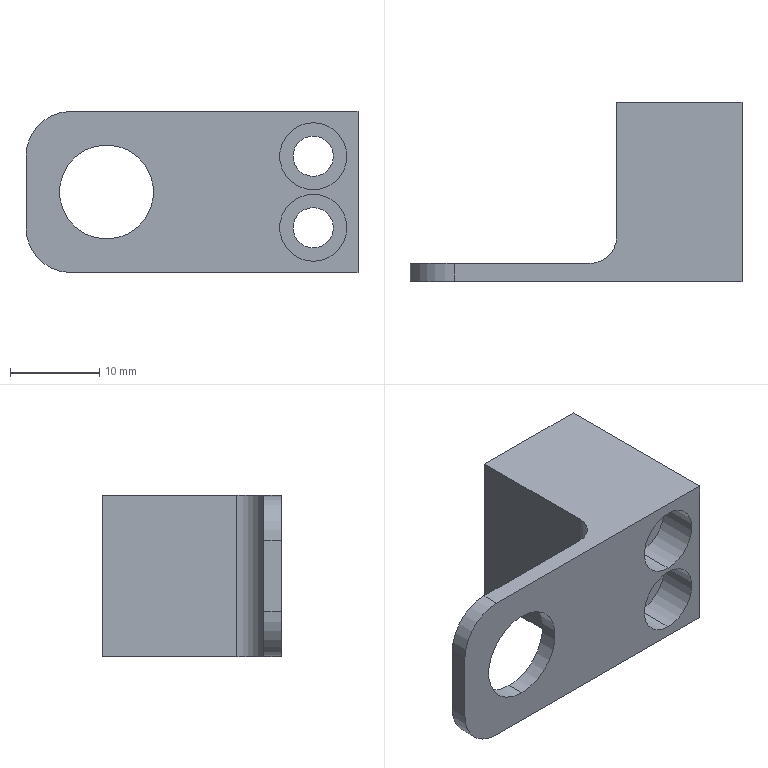Component | SolidWorks | 7.1.02.0001.00.00-0050-1 | 1 solid | 23 faces | box 37.1 x 20 x 18 mm | volume 4827 mm3 | cylinder 13 | plane 10 | commonest cylinder face diameters 7.5 x4 4.5 x4 10.5 x2 10 x2 6 x1
build123d program:
from build123d import *

# Parameters (mm, degrees)
BOSS_EXTRUDE1_DEPTH                             = 9
M4_HEX_SOCKET_HEAD_CAP_SCREW_CBORE1_D           = 4.5
M4_HEX_SOCKET_HEAD_CAP_SCREW_CBORE1_CBORE_D     = 7.5
M4_HEX_SOCKET_HEAD_CAP_SCREW_CBORE1_CBORE_DEPTH = 4.4
SKETCH3_R                                       = 5.25
CUT_EXTRUDE1_DEPTH                              = 29.725
FILLET1_R                                       = 5


with BuildPart() as part:
    # Sketch1 → Boss-Extrude1 (new, symmetric)
    with BuildSketch(Plane.XY):
        with BuildLine():
            Line((8, 18.55), (8, -1.55))
            ThreePointArc((8, -1.55), (7.121, -3.671), (5, -4.55))
            Line((5, -4.55), (-10, -4.55))
            Line((-10, -4.55), (-10, -18.55))
            Line((-10, -18.55), (10, -18.55))
            Line((10, -18.55), (10, 18.55))
            Line((10, 18.55), (8, 18.55))
        make_face()
    extrude(amount=BOSS_EXTRUDE1_DEPTH, both=True)

    # M4 Hex Socket Head Cap Screw CBORE1 (through all)
    with Locations(Plane(origin=(10, -13.55, -4), x_dir=(0, 0, 1), z_dir=(1, 0, 0))):
        with Locations((0, 0), (8, 0)):
            CounterBoreHole(M4_HEX_SOCKET_HEAD_CAP_SCREW_CBORE1_D / 2, M4_HEX_SOCKET_HEAD_CAP_SCREW_CBORE1_CBORE_D / 2, M4_HEX_SOCKET_HEAD_CAP_SCREW_CBORE1_CBORE_DEPTH)

    # Sketch3 → Cut-Extrude1 (cut, through all)
    with BuildSketch(Plane(origin=(10, 0, 0), x_dir=(0, 0, -1), z_dir=(1, 0, 0))):
        with Locations((0, 9.55)):
            Circle(SKETCH3_R)
    extrude(amount=-CUT_EXTRUDE1_DEPTH, mode=Mode.SUBTRACT)

    # Fillet1
    fillet1_edges = [part.edges().sort_by_distance(p)[0] for p in [
        (9, 18.55, 9),
        (9, 18.55, -9),
    ]]
    fillet(fillet1_edges, radius=FILLET1_R)


solid = part.part

# Placed as in the assembly
solid = solid.moved(Location((-44.514, -58.684, 0), (180, 0, 90)))
STEP:
#1=CARTESIAN_POINT('',(-2.128,-2.625,-0.2067));
#2=VERTEX_POINT('',#1);
#3=CARTESIAN_POINT('',(-2.128,-2.625,0.2067));
#4=VERTEX_POINT('',#3);
#5=CARTESIAN_POINT('',(-2.128,-2.625,-0.));
#6=DIRECTION('',(-0.,-1.,-0.));
#7=DIRECTION('',(-1.,0.,0.));
#8=AXIS2_PLACEMENT_3D('',#5,#6,#7);
#9=CIRCLE('',#8,0.2067);
#10=EDGE_CURVE('',#2,#4,#9,.T.);
#11=ORIENTED_EDGE('',*,*,#10,.F.);
#12=CARTESIAN_POINT('',(-2.128,-2.704,-0.2067));
#13=VERTEX_POINT('',#12);
#14=CARTESIAN_POINT('',(-2.128,-1.917,-0.2067));
#15=DIRECTION('',(-0.,-1.,-0.));
#16=VECTOR('',#15,39.37);
#17=LINE('',#14,#16);
#18=EDGE_CURVE('',#2,#13,#17,.T.);
#19=ORIENTED_EDGE('',*,*,#18,.T.);
#20=CARTESIAN_POINT('',(-2.128,-2.704,0.2067));
#21=VERTEX_POINT('',#20);
#22=CARTESIAN_POINT('',(-2.128,-2.704,-0.));
#23=DIRECTION('',(-0.,-1.,-0.));
#24=DIRECTION('',(0.,0.,1.));
#25=AXIS2_PLACEMENT_3D('',#22,#23,#24);
#26=CIRCLE('',#25,0.2067);
#27=EDGE_CURVE('',#13,#21,#26,.T.);
#28=ORIENTED_EDGE('',*,*,#27,.T.);
#29=CARTESIAN_POINT('',(-2.128,-1.917,0.2067));
#30=DIRECTION('',(-0.,-1.,-0.));
#31=VECTOR('',#30,39.37);
#32=LINE('',#29,#31);
#33=EDGE_CURVE('',#4,#21,#32,.T.);
#34=ORIENTED_EDGE('',*,*,#33,.F.);
#35=EDGE_LOOP('',(#11,#19,#28,#34));
#36=FACE_OUTER_BOUND('',#35,.T.);
#37=CARTESIAN_POINT('',(-2.128,-1.917,-0.));
#38=DIRECTION('',(-0.,-1.,-0.));
#39=DIRECTION('',(0.,0.,1.));
#40=AXIS2_PLACEMENT_3D('',#37,#38,#39);
#41=CYLINDRICAL_SURFACE('',#40,0.2067);
#42=ADVANCED_FACE('',(#36),#41,.F.);
#43=CARTESIAN_POINT('',(-1.219,-2.531,0.009843));
#44=VERTEX_POINT('',#43);
#45=CARTESIAN_POINT('',(-1.219,-2.531,0.3051));
#46=VERTEX_POINT('',#45);
#47=CARTESIAN_POINT('',(-1.219,-2.531,0.1575));
#48=DIRECTION('',(-0.,-1.,-0.));
#49=DIRECTION('',(0.,0.,1.));
#50=AXIS2_PLACEMENT_3D('',#47,#48,#49);
#51=CIRCLE('',#50,0.1476);
#52=EDGE_CURVE('',#44,#46,#51,.T.);
#53=ORIENTED_EDGE('',*,*,#52,.F.);
#54=CARTESIAN_POINT('',(-1.219,-2.704,0.009843));
#55=VERTEX_POINT('',#54);
#56=CARTESIAN_POINT('',(-1.219,-2.704,0.009843));
#57=DIRECTION('',(-0.,-1.,-0.));
#58=VECTOR('',#57,39.37);
#59=LINE('',#56,#58);
#60=EDGE_CURVE('',#44,#55,#59,.T.);
#61=ORIENTED_EDGE('',*,*,#60,.T.);
#62=CARTESIAN_POINT('',(-1.219,-2.704,0.3051));
#63=VERTEX_POINT('',#62);
#64=CARTESIAN_POINT('',(-1.219,-2.704,0.1575));
#65=DIRECTION('',(-0.,-1.,-0.));
#66=DIRECTION('',(0.,0.,1.));
#67=AXIS2_PLACEMENT_3D('',#64,#65,#66);
#68=CIRCLE('',#67,0.1476);
#69=EDGE_CURVE('',#55,#63,#68,.T.);
#70=ORIENTED_EDGE('',*,*,#69,.T.);
#71=CARTESIAN_POINT('',(-1.219,-2.704,0.3051));
#72=DIRECTION('',(-0.,-1.,-0.));
#73=VECTOR('',#72,39.37);
#74=LINE('',#71,#73);
#75=EDGE_CURVE('',#46,#63,#74,.T.);
#76=ORIENTED_EDGE('',*,*,#75,.F.);
#77=EDGE_LOOP('',(#53,#61,#70,#76));
#78=FACE_OUTER_BOUND('',#77,.T.);
#79=CARTESIAN_POINT('',(-1.219,-2.704,0.1575));
#80=DIRECTION('',(-0.,-1.,-0.));
#81=DIRECTION('',(0.,0.,1.));
#82=AXIS2_PLACEMENT_3D('',#79,#80,#81);
#83=CYLINDRICAL_SURFACE('',#82,0.1476);
#84=ADVANCED_FACE('',(#78),#83,.F.);
#85=CARTESIAN_POINT('',(-1.219,-1.917,0.0689));
#86=VERTEX_POINT('',#85);
#87=CARTESIAN_POINT('',(-1.219,-1.917,0.2461));
#88=VERTEX_POINT('',#87);
#89=CARTESIAN_POINT('',(-1.219,-1.917,0.1575));
#90=DIRECTION('',(-0.,-1.,-0.));
#91=DIRECTION('',(0.,0.,1.));
#92=AXIS2_PLACEMENT_3D('',#89,#90,#91);
#93=CIRCLE('',#92,0.08858);
#94=EDGE_CURVE('',#86,#88,#93,.T.);
#95=ORIENTED_EDGE('',*,*,#94,.F.);
#96=CARTESIAN_POINT('',(-1.219,-2.531,0.0689));
#97=VERTEX_POINT('',#96);
#98=CARTESIAN_POINT('',(-1.219,-2.704,0.0689));
#99=DIRECTION('',(-0.,-1.,-0.));
#100=VECTOR('',#99,39.37);
#101=LINE('',#98,#100);
#102=EDGE_CURVE('',#86,#97,#101,.T.);
#103=ORIENTED_EDGE('',*,*,#102,.T.);
#104=CARTESIAN_POINT('',(-1.219,-2.531,0.2461));
#105=VERTEX_POINT('',#104);
#106=CARTESIAN_POINT('',(-1.219,-2.531,0.1575));
#107=DIRECTION('',(-0.,-1.,-0.));
#108=DIRECTION('',(0.,0.,1.));
#109=AXIS2_PLACEMENT_3D('',#106,#107,#108);
#110=CIRCLE('',#109,0.08858);
#111=EDGE_CURVE('',#97,#105,#110,.T.);
#112=ORIENTED_EDGE('',*,*,#111,.T.);
#113=CARTESIAN_POINT('',(-1.219,-2.704,0.2461));
#114=DIRECTION('',(-0.,-1.,-0.));
#115=VECTOR('',#114,39.37);
#116=LINE('',#113,#115);
#117=EDGE_CURVE('',#88,#105,#116,.T.);
#118=ORIENTED_EDGE('',*,*,#117,.F.);
#119=EDGE_LOOP('',(#95,#103,#112,#118));
#120=FACE_OUTER_BOUND('',#119,.T.);
#121=CARTESIAN_POINT('',(-1.219,-2.704,0.1575));
#122=DIRECTION('',(-0.,-1.,-0.));
#123=DIRECTION('',(0.,0.,1.));
#124=AXIS2_PLACEMENT_3D('',#121,#122,#123);
#125=CYLINDRICAL_SURFACE('',#124,0.08858);
#126=ADVANCED_FACE('',(#120),#125,.F.);
#127=CARTESIAN_POINT('',(-1.219,-2.531,-0.3051));
#128=VERTEX_POINT('',#127);
#129=CARTESIAN_POINT('',(-1.219,-2.531,-0.009843));
#130=VERTEX_POINT('',#129);
#131=CARTESIAN_POINT('',(-1.219,-2.531,-0.1575));
#132=DIRECTION('',(-0.,-1.,-0.));
#133=DIRECTION('',(0.,0.,1.));
#134=AXIS2_PLACEMENT_3D('',#131,#132,#133);
#135=CIRCLE('',#134,0.1476);
#136=EDGE_CURVE('',#128,#130,#135,.T.);
#137=ORIENTED_EDGE('',*,*,#136,.F.);
#138=CARTESIAN_POINT('',(-1.219,-2.704,-0.3051));
#139=VERTEX_POINT('',#138);
#140=CARTESIAN_POINT('',(-1.219,-2.704,-0.3051));
#141=DIRECTION('',(-0.,-1.,-0.));
#142=VECTOR('',#141,39.37);
#143=LINE('',#140,#142);
#144=EDGE_CURVE('',#128,#139,#143,.T.);
#145=ORIENTED_EDGE('',*,*,#144,.T.);
#146=CARTESIAN_POINT('',(-1.219,-2.704,-0.009843));
#147=VERTEX_POINT('',#146);
#148=CARTESIAN_POINT('',(-1.219,-2.704,-0.1575));
#149=DIRECTION('',(-0.,-1.,-0.));
#150=DIRECTION('',(0.,0.,1.));
#151=AXIS2_PLACEMENT_3D('',#148,#149,#150);
#152=CIRCLE('',#151,0.1476);
#153=EDGE_CURVE('',#139,#147,#152,.T.);
#154=ORIENTED_EDGE('',*,*,#153,.T.);
#155=CARTESIAN_POINT('',(-1.219,-2.704,-0.009843));
#156=DIRECTION('',(-0.,-1.,-0.));
#157=VECTOR('',#156,39.37);
#158=LINE('',#155,#157);
#159=EDGE_CURVE('',#130,#147,#158,.T.);
#160=ORIENTED_EDGE('',*,*,#159,.F.);
#161=EDGE_LOOP('',(#137,#145,#154,#160));
#162=FACE_OUTER_BOUND('',#161,.T.);
#163=CARTESIAN_POINT('',(-1.219,-2.704,-0.1575));
#164=DIRECTION('',(-0.,-1.,-0.));
#165=DIRECTION('',(0.,0.,1.));
#166=AXIS2_PLACEMENT_3D('',#163,#164,#165);
#167=CYLINDRICAL_SURFACE('',#166,0.1476);
#168=ADVANCED_FACE('',(#162),#167,.F.);
#169=CARTESIAN_POINT('',(-1.219,-1.917,-0.2461));
#170=VERTEX_POINT('',#169);
#171=CARTESIAN_POINT('',(-1.219,-1.917,-0.0689));
#172=VERTEX_POINT('',#171);
#173=CARTESIAN_POINT('',(-1.219,-1.917,-0.1575));
#174=DIRECTION('',(-0.,-1.,-0.));
#175=DIRECTION('',(0.,0.,1.));
#176=AXIS2_PLACEMENT_3D('',#173,#174,#175);
#177=CIRCLE('',#176,0.08858);
#178=EDGE_CURVE('',#170,#172,#177,.T.);
#179=ORIENTED_EDGE('',*,*,#178,.F.);
#180=CARTESIAN_POINT('',(-1.219,-2.531,-0.2461));
#181=VERTEX_POINT('',#180);
#182=CARTESIAN_POINT('',(-1.219,-2.704,-0.2461));
#183=DIRECTION('',(-0.,-1.,-0.));
#184=VECTOR('',#183,39.37);
#185=LINE('',#182,#184);
#186=EDGE_CURVE('',#170,#181,#185,.T.);
#187=ORIENTED_EDGE('',*,*,#186,.T.);
#188=CARTESIAN_POINT('',(-1.219,-2.531,-0.0689));
#189=VERTEX_POINT('',#188);
#190=CARTESIAN_POINT('',(-1.219,-2.531,-0.1575));
#191=DIRECTION('',(-0.,-1.,-0.));
#192=DIRECTION('',(0.,0.,1.));
#193=AXIS2_PLACEMENT_3D('',#190,#191,#192);
#194=CIRCLE('',#193,0.08858);
#195=EDGE_CURVE('',#181,#189,#194,.T.);
#196=ORIENTED_EDGE('',*,*,#195,.T.);
#197=CARTESIAN_POINT('',(-1.219,-2.704,-0.0689));
#198=DIRECTION('',(-0.,-1.,-0.));
#199=VECTOR('',#198,39.37);
#200=LINE('',#197,#199);
#201=EDGE_CURVE('',#172,#189,#200,.T.);
#202=ORIENTED_EDGE('',*,*,#201,.F.);
#203=EDGE_LOOP('',(#179,#187,#196,#202));
#204=FACE_OUTER_BOUND('',#203,.T.);
#205=CARTESIAN_POINT('',(-1.219,-2.704,-0.1575));
#206=DIRECTION('',(-0.,-1.,-0.));
#207=DIRECTION('',(0.,0.,1.));
#208=AXIS2_PLACEMENT_3D('',#205,#206,#207);
#209=CYLINDRICAL_SURFACE('',#208,0.08858);
#210=ADVANCED_FACE('',(#204),#209,.F.);
#211=CARTESIAN_POINT('',(-1.691,-2.625,0.3543));
#212=VERTEX_POINT('',#211);
#213=CARTESIAN_POINT('',(-1.573,-2.507,0.3543));
#214=VERTEX_POINT('',#213);
#215=CARTESIAN_POINT('',(-1.691,-2.507,0.3543));
#216=DIRECTION('',(0.,-0.,1.));
#217=DIRECTION('',(0.,1.,0.));
#218=AXIS2_PLACEMENT_3D('',#215,#216,#217);
#219=CIRCLE('',#218,0.1181);
#220=EDGE_CURVE('',#212,#214,#219,.T.);
#221=ORIENTED_EDGE('',*,*,#220,.T.);
#222=CARTESIAN_POINT('',(-1.573,-2.507,-0.3543));
#223=VERTEX_POINT('',#222);
#224=CARTESIAN_POINT('',(-1.573,-2.507,-0.3543));
#225=DIRECTION('',(0.,-0.,1.));
#226=VECTOR('',#225,39.37);
#227=LINE('',#224,#226);
#228=EDGE_CURVE('',#223,#214,#227,.T.);
#229=ORIENTED_EDGE('',*,*,#228,.F.);
#230=CARTESIAN_POINT('',(-1.691,-2.625,-0.3543));
#231=VERTEX_POINT('',#230);
#232=CARTESIAN_POINT('',(-1.691,-2.507,-0.3543));
#233=DIRECTION('',(0.,-0.,1.));
#234=DIRECTION('',(0.,1.,0.));
#235=AXIS2_PLACEMENT_3D('',#232,#233,#234);
#236=CIRCLE('',#235,0.1181);
#237=EDGE_CURVE('',#231,#223,#236,.T.);
#238=ORIENTED_EDGE('',*,*,#237,.F.);
#239=CARTESIAN_POINT('',(-1.691,-2.625,-0.3543));
#240=DIRECTION('',(0.,-0.,1.));
#241=VECTOR('',#240,39.37);
#242=LINE('',#239,#241);
#243=EDGE_CURVE('',#231,#212,#242,.T.);
#244=ORIENTED_EDGE('',*,*,#243,.T.);
#245=EDGE_LOOP('',(#221,#229,#238,#244));
#246=FACE_OUTER_BOUND('',#245,.T.);
#247=CARTESIAN_POINT('',(-1.691,-2.507,-0.3543));
#248=DIRECTION('',(0.,-0.,1.));
#249=DIRECTION('',(0.,1.,0.));
#250=AXIS2_PLACEMENT_3D('',#247,#248,#249);
#251=CYLINDRICAL_SURFACE('',#250,0.1181);
#252=ADVANCED_FACE('',(#246),#251,.F.);
#253=CARTESIAN_POINT('',(-1.573,-1.917,0.3543));
#254=VERTEX_POINT('',#253);
#255=CARTESIAN_POINT('',(-1.573,-2.507,0.3543));
#256=DIRECTION('',(0.,1.,0.));
#257=VECTOR('',#256,39.37);
#258=LINE('',#255,#257);
#259=EDGE_CURVE('',#214,#254,#258,.T.);
#260=ORIENTED_EDGE('',*,*,#259,.T.);
#261=CARTESIAN_POINT('',(-1.573,-1.917,-0.3543));
#262=VERTEX_POINT('',#261);
#263=CARTESIAN_POINT('',(-1.573,-1.917,-0.3543));
#264=DIRECTION('',(0.,-0.,1.));
#265=VECTOR('',#264,39.37);
#266=LINE('',#263,#265);
#267=EDGE_CURVE('',#262,#254,#266,.T.);
#268=ORIENTED_EDGE('',*,*,#267,.F.);
#269=CARTESIAN_POINT('',(-1.573,-2.507,-0.3543));
#270=DIRECTION('',(0.,1.,0.));
#271=VECTOR('',#270,39.37);
#272=LINE('',#269,#271);
#273=EDGE_CURVE('',#223,#262,#272,.T.);
#274=ORIENTED_EDGE('',*,*,#273,.F.);
#275=ORIENTED_EDGE('',*,*,#228,.T.);
#276=EDGE_LOOP('',(#260,#268,#274,#275));
#277=FACE_OUTER_BOUND('',#276,.T.);
#278=CARTESIAN_POINT('',(-1.573,-2.507,-0.3543));
#279=DIRECTION('',(1.,-0.,-0.));
#280=DIRECTION('',(-0.,-1.,-0.));
#281=AXIS2_PLACEMENT_3D('',#278,#279,#280);
#282=PLANE('',#281);
#283=ADVANCED_FACE('',(#277),#282,.F.);
#284=CARTESIAN_POINT('',(-1.219,-1.917,0.1575));
#285=DIRECTION('',(-0.,-1.,-0.));
#286=DIRECTION('',(0.,0.,1.));
#287=AXIS2_PLACEMENT_3D('',#284,#285,#286);
#288=CIRCLE('',#287,0.08858);
#289=EDGE_CURVE('',#88,#86,#288,.T.);
#290=ORIENTED_EDGE('',*,*,#289,.T.);
#291=ORIENTED_EDGE('',*,*,#94,.T.);
#292=EDGE_LOOP('',(#290,#291));
#293=FACE_BOUND('',#292,.T.);
#294=CARTESIAN_POINT('',(-1.219,-1.917,-0.1575));
#295=DIRECTION('',(-0.,-1.,-0.));
#296=DIRECTION('',(0.,0.,1.));
#297=AXIS2_PLACEMENT_3D('',#294,#295,#296);
#298=CIRCLE('',#297,0.08858);
#299=EDGE_CURVE('',#172,#170,#298,.T.);
#300=ORIENTED_EDGE('',*,*,#299,.T.);
#301=ORIENTED_EDGE('',*,*,#178,.T.);
#302=EDGE_LOOP('',(#300,#301));
#303=FACE_BOUND('',#302,.T.);
#304=CARTESIAN_POINT('',(-1.022,-1.917,0.3543));
#305=VERTEX_POINT('',#304);
#306=CARTESIAN_POINT('',(-1.573,-1.917,0.3543));
#307=DIRECTION('',(1.,0.,-0.));
#308=VECTOR('',#307,39.37);
#309=LINE('',#306,#308);
#310=EDGE_CURVE('',#254,#305,#309,.T.);
#311=ORIENTED_EDGE('',*,*,#310,.T.);
#312=CARTESIAN_POINT('',(-1.022,-1.917,-0.3543));
#313=VERTEX_POINT('',#312);
#314=CARTESIAN_POINT('',(-1.022,-1.917,-0.3543));
#315=DIRECTION('',(0.,-0.,1.));
#316=VECTOR('',#315,39.37);
#317=LINE('',#314,#316);
#318=EDGE_CURVE('',#313,#305,#317,.T.);
#319=ORIENTED_EDGE('',*,*,#318,.F.);
#320=CARTESIAN_POINT('',(-1.573,-1.917,-0.3543));
#321=DIRECTION('',(1.,0.,-0.));
#322=VECTOR('',#321,39.37);
#323=LINE('',#320,#322);
#324=EDGE_CURVE('',#262,#313,#323,.T.);
#325=ORIENTED_EDGE('',*,*,#324,.F.);
#326=ORIENTED_EDGE('',*,*,#267,.T.);
#327=EDGE_LOOP('',(#311,#319,#325,#326));
#328=FACE_OUTER_BOUND('',#327,.T.);
#329=CARTESIAN_POINT('',(-1.573,-1.917,-0.3543));
#330=DIRECTION('',(0.,-1.,-0.));
#331=DIRECTION('',(-1.,-0.,0.));
#332=AXIS2_PLACEMENT_3D('',#329,#330,#331);
#333=PLANE('',#332);
#334=ADVANCED_FACE('',(#293,#303,#328),#333,.F.);
#335=CARTESIAN_POINT('',(-1.022,-2.704,0.3543));
#336=VERTEX_POINT('',#335);
#337=CARTESIAN_POINT('',(-1.022,-1.917,0.3543));
#338=DIRECTION('',(-0.,-1.,-0.));
#339=VECTOR('',#338,39.37);
#340=LINE('',#337,#339);
#341=EDGE_CURVE('',#305,#336,#340,.T.);
#342=ORIENTED_EDGE('',*,*,#341,.T.);
#343=CARTESIAN_POINT('',(-1.022,-2.704,-0.3543));
#344=VERTEX_POINT('',#343);
#345=CARTESIAN_POINT('',(-1.022,-2.704,-0.3543));
#346=DIRECTION('',(0.,-0.,1.));
#347=VECTOR('',#346,39.37);
#348=LINE('',#345,#347);
#349=EDGE_CURVE('',#344,#336,#348,.T.);
#350=ORIENTED_EDGE('',*,*,#349,.F.);
#351=CARTESIAN_POINT('',(-1.022,-1.917,-0.3543));
#352=DIRECTION('',(-0.,-1.,-0.));
#353=VECTOR('',#352,39.37);
#354=LINE('',#351,#353);
#355=EDGE_CURVE('',#313,#344,#354,.T.);
#356=ORIENTED_EDGE('',*,*,#355,.F.);
#357=ORIENTED_EDGE('',*,*,#318,.T.);
#358=EDGE_LOOP('',(#342,#350,#356,#357));
#359=FACE_OUTER_BOUND('',#358,.T.);
#360=CARTESIAN_POINT('',(-1.022,-1.917,-0.3543));
#361=DIRECTION('',(-1.,0.,0.));
#362=DIRECTION('',(-0.,0.,-1.));
#363=AXIS2_PLACEMENT_3D('',#360,#361,#362);
#364=PLANE('',#363);
#365=ADVANCED_FACE('',(#359),#364,.F.);
#366=CARTESIAN_POINT('',(-2.128,-2.704,-0.));
#367=DIRECTION('',(-0.,-1.,-0.));
#368=DIRECTION('',(0.,0.,1.));
#369=AXIS2_PLACEMENT_3D('',#366,#367,#368);
#370=CIRCLE('',#369,0.2067);
#371=EDGE_CURVE('',#21,#13,#370,.T.);
#372=ORIENTED_EDGE('',*,*,#371,.F.);
#373=ORIENTED_EDGE('',*,*,#27,.F.);
#374=EDGE_LOOP('',(#372,#373));
#375=FACE_BOUND('',#374,.T.);
#376=CARTESIAN_POINT('',(-1.219,-2.704,0.1575));
#377=DIRECTION('',(-0.,-1.,-0.));
#378=DIRECTION('',(0.,0.,1.));
#379=AXIS2_PLACEMENT_3D('',#376,#377,#378);
#380=CIRCLE('',#379,0.1476);
#381=EDGE_CURVE('',#63,#55,#380,.T.);
#382=ORIENTED_EDGE('',*,*,#381,.F.);
#383=ORIENTED_EDGE('',*,*,#69,.F.);
#384=EDGE_LOOP('',(#382,#383));
#385=FACE_BOUND('',#384,.T.);
#386=CARTESIAN_POINT('',(-1.219,-2.704,-0.1575));
#387=DIRECTION('',(-0.,-1.,-0.));
#388=DIRECTION('',(0.,0.,1.));
#389=AXIS2_PLACEMENT_3D('',#386,#387,#388);
#390=CIRCLE('',#389,0.1476);
#391=EDGE_CURVE('',#147,#139,#390,.T.);
#392=ORIENTED_EDGE('',*,*,#391,.F.);
#393=ORIENTED_EDGE('',*,*,#153,.F.);
#394=EDGE_LOOP('',(#392,#393));
#395=FACE_BOUND('',#394,.T.);
#396=CARTESIAN_POINT('',(-2.286,-2.704,0.3543));
#397=VERTEX_POINT('',#396);
#398=CARTESIAN_POINT('',(-2.483,-2.704,0.3543));
#399=DIRECTION('',(-1.,0.,0.));
#400=VECTOR('',#399,39.37);
#401=LINE('',#398,#400);
#402=EDGE_CURVE('',#336,#397,#401,.T.);
#403=ORIENTED_EDGE('',*,*,#402,.T.);
#404=CARTESIAN_POINT('',(-2.483,-2.704,0.1575));
#405=VERTEX_POINT('',#404);
#406=CARTESIAN_POINT('',(-2.286,-2.704,0.1575));
#407=DIRECTION('',(-0.,-1.,-0.));
#408=DIRECTION('',(0.,0.,-1.));
#409=AXIS2_PLACEMENT_3D('',#406,#407,#408);
#410=CIRCLE('',#409,0.1969);
#411=EDGE_CURVE('',#397,#405,#410,.T.);
#412=ORIENTED_EDGE('',*,*,#411,.T.);
#413=CARTESIAN_POINT('',(-2.483,-2.704,-0.1575));
#414=VERTEX_POINT('',#413);
#415=CARTESIAN_POINT('',(-2.483,-2.704,-0.3543));
#416=DIRECTION('',(0.,-0.,1.));
#417=VECTOR('',#416,39.37);
#418=LINE('',#415,#417);
#419=EDGE_CURVE('',#414,#405,#418,.T.);
#420=ORIENTED_EDGE('',*,*,#419,.F.);
#421=CARTESIAN_POINT('',(-2.286,-2.704,-0.3543));
#422=VERTEX_POINT('',#421);
#423=CARTESIAN_POINT('',(-2.286,-2.704,-0.1575));
#424=DIRECTION('',(-0.,-1.,-0.));
#425=DIRECTION('',(0.,0.,-1.));
#426=AXIS2_PLACEMENT_3D('',#423,#424,#425);
#427=CIRCLE('',#426,0.1969);
#428=EDGE_CURVE('',#414,#422,#427,.T.);
#429=ORIENTED_EDGE('',*,*,#428,.T.);
#430=CARTESIAN_POINT('',(-2.483,-2.704,-0.3543));
#431=DIRECTION('',(-1.,0.,0.));
#432=VECTOR('',#431,39.37);
#433=LINE('',#430,#432);
#434=EDGE_CURVE('',#344,#422,#433,.T.);
#435=ORIENTED_EDGE('',*,*,#434,.F.);
#436=ORIENTED_EDGE('',*,*,#349,.T.);
#437=EDGE_LOOP('',(#403,#412,#420,#429,#435,#436));
#438=FACE_OUTER_BOUND('',#437,.T.);
#439=CARTESIAN_POINT('',(-2.483,-2.704,-0.3543));
#440=DIRECTION('',(0.,1.,0.));
#441=DIRECTION('',(-0.,0.,-1.));
#442=AXIS2_PLACEMENT_3D('',#439,#440,#441);
#443=PLANE('',#442);
#444=ADVANCED_FACE('',(#375,#385,#395,#438),#443,.F.);
#445=ORIENTED_EDGE('',*,*,#419,.T.);
#446=CARTESIAN_POINT('',(-2.483,-2.625,0.1575));
#447=VERTEX_POINT('',#446);
#448=CARTESIAN_POINT('',(-2.483,-2.625,0.1575));
#449=DIRECTION('',(0.,1.,0.));
#450=VECTOR('',#449,39.37);
#451=LINE('',#448,#450);
#452=EDGE_CURVE('',#405,#447,#451,.T.);
#453=ORIENTED_EDGE('',*,*,#452,.T.);
#454=CARTESIAN_POINT('',(-2.483,-2.625,-0.1575));
#455=VERTEX_POINT('',#454);
#456=CARTESIAN_POINT('',(-2.483,-2.625,-0.3543));
#457=DIRECTION('',(0.,-0.,1.));
#458=VECTOR('',#457,39.37);
#459=LINE('',#456,#458);
#460=EDGE_CURVE('',#455,#447,#459,.T.);
#461=ORIENTED_EDGE('',*,*,#460,.F.);
#462=CARTESIAN_POINT('',(-2.483,-2.625,-0.1575));
#463=DIRECTION('',(-0.,-1.,-0.));
#464=VECTOR('',#463,39.37);
#465=LINE('',#462,#464);
#466=EDGE_CURVE('',#455,#414,#465,.T.);
#467=ORIENTED_EDGE('',*,*,#466,.T.);
#468=EDGE_LOOP('',(#445,#453,#461,#467));
#469=FACE_OUTER_BOUND('',#468,.T.);
#470=CARTESIAN_POINT('',(-2.483,-2.625,-0.3543));
#471=DIRECTION('',(1.,-0.,-0.));
#472=DIRECTION('',(0.,-0.,1.));
#473=AXIS2_PLACEMENT_3D('',#470,#471,#472);
#474=PLANE('',#473);
#475=ADVANCED_FACE('',(#469),#474,.F.);
#476=CARTESIAN_POINT('',(-2.128,-2.625,-0.));
#477=DIRECTION('',(-0.,-1.,-0.));
#478=DIRECTION('',(-1.,0.,0.));
#479=AXIS2_PLACEMENT_3D('',#476,#477,#478);
#480=CIRCLE('',#479,0.2067);
#481=EDGE_CURVE('',#4,#2,#480,.T.);
#482=ORIENTED_EDGE('',*,*,#481,.T.);
#483=ORIENTED_EDGE('',*,*,#10,.T.);
#484=EDGE_LOOP('',(#482,#483));
#485=FACE_BOUND('',#484,.T.);
#486=ORIENTED_EDGE('',*,*,#460,.T.);
#487=CARTESIAN_POINT('',(-2.286,-2.625,0.3543));
#488=VERTEX_POINT('',#487);
#489=CARTESIAN_POINT('',(-2.286,-2.625,0.1575));
#490=DIRECTION('',(0.,1.,0.));
#491=DIRECTION('',(-1.,0.,0.));
#492=AXIS2_PLACEMENT_3D('',#489,#490,#491);
#493=CIRCLE('',#492,0.1969);
#494=EDGE_CURVE('',#447,#488,#493,.T.);
#495=ORIENTED_EDGE('',*,*,#494,.T.);
#496=CARTESIAN_POINT('',(-2.483,-2.625,0.3543));
#497=DIRECTION('',(1.,-0.,-0.));
#498=VECTOR('',#497,39.37);
#499=LINE('',#496,#498);
#500=EDGE_CURVE('',#488,#212,#499,.T.);
#501=ORIENTED_EDGE('',*,*,#500,.T.);
#502=ORIENTED_EDGE('',*,*,#243,.F.);
#503=CARTESIAN_POINT('',(-2.286,-2.625,-0.3543));
#504=VERTEX_POINT('',#503);
#505=CARTESIAN_POINT('',(-2.483,-2.625,-0.3543));
#506=DIRECTION('',(1.,-0.,-0.));
#507=VECTOR('',#506,39.37);
#508=LINE('',#505,#507);
#509=EDGE_CURVE('',#504,#231,#508,.T.);
#510=ORIENTED_EDGE('',*,*,#509,.F.);
#511=CARTESIAN_POINT('',(-2.286,-2.625,-0.1575));
#512=DIRECTION('',(0.,1.,0.));
#513=DIRECTION('',(-1.,0.,0.));
#514=AXIS2_PLACEMENT_3D('',#511,#512,#513);
#515=CIRCLE('',#514,0.1969);
#516=EDGE_CURVE('',#504,#455,#515,.T.);
#517=ORIENTED_EDGE('',*,*,#516,.T.);
#518=EDGE_LOOP('',(#486,#495,#501,#502,#510,#517));
#519=FACE_OUTER_BOUND('',#518,.T.);
#520=CARTESIAN_POINT('',(-2.483,-2.625,-0.3543));
#521=DIRECTION('',(-0.,-1.,-0.));
#522=DIRECTION('',(-1.,0.,0.));
#523=AXIS2_PLACEMENT_3D('',#520,#521,#522);
#524=PLANE('',#523);
#525=ADVANCED_FACE('',(#485,#519),#524,.F.);
#526=ORIENTED_EDGE('',*,*,#434,.T.);
#527=CARTESIAN_POINT('',(-2.286,-2.507,-0.3543));
#528=DIRECTION('',(0.,1.,0.));
#529=VECTOR('',#528,39.37);
#530=LINE('',#527,#529);
#531=EDGE_CURVE('',#422,#504,#530,.T.);
#532=ORIENTED_EDGE('',*,*,#531,.T.);
#533=ORIENTED_EDGE('',*,*,#509,.T.);
#534=ORIENTED_EDGE('',*,*,#237,.T.);
#535=ORIENTED_EDGE('',*,*,#273,.T.);
#536=ORIENTED_EDGE('',*,*,#324,.T.);
#537=ORIENTED_EDGE('',*,*,#355,.T.);
#538=EDGE_LOOP('',(#526,#532,#533,#534,#535,#536,#537));
#539=FACE_OUTER_BOUND('',#538,.T.);
#540=CARTESIAN_POINT('',(-1.691,-2.507,-0.3543));
#541=DIRECTION('',(0.,-0.,1.));
#542=DIRECTION('',(0.,1.,0.));
#543=AXIS2_PLACEMENT_3D('',#540,#541,#542);
#544=PLANE('',#543);
#545=ADVANCED_FACE('',(#539),#544,.F.);
#546=ORIENTED_EDGE('',*,*,#500,.F.);
#547=CARTESIAN_POINT('',(-2.286,-2.704,0.3543));
#548=DIRECTION('',(-0.,-1.,-0.));
#549=VECTOR('',#548,39.37);
#550=LINE('',#547,#549);
#551=EDGE_CURVE('',#488,#397,#550,.T.);
#552=ORIENTED_EDGE('',*,*,#551,.T.);
#553=ORIENTED_EDGE('',*,*,#402,.F.);
#554=ORIENTED_EDGE('',*,*,#341,.F.);
#555=ORIENTED_EDGE('',*,*,#310,.F.);
#556=ORIENTED_EDGE('',*,*,#259,.F.);
#557=ORIENTED_EDGE('',*,*,#220,.F.);
#558=EDGE_LOOP('',(#546,#552,#553,#554,#555,#556,#557));
#559=FACE_OUTER_BOUND('',#558,.T.);
#560=CARTESIAN_POINT('',(-1.691,-2.507,0.3543));
#561=DIRECTION('',(0.,-0.,1.));
#562=DIRECTION('',(0.,1.,0.));
#563=AXIS2_PLACEMENT_3D('',#560,#561,#562);
#564=PLANE('',#563);
#565=ADVANCED_FACE('',(#559),#564,.T.);
#566=ORIENTED_EDGE('',*,*,#186,.F.);
#567=ORIENTED_EDGE('',*,*,#299,.F.);
#568=ORIENTED_EDGE('',*,*,#201,.T.);
#569=CARTESIAN_POINT('',(-1.219,-2.531,-0.1575));
#570=DIRECTION('',(-0.,-1.,-0.));
#571=DIRECTION('',(0.,0.,1.));
#572=AXIS2_PLACEMENT_3D('',#569,#570,#571);
#573=CIRCLE('',#572,0.08858);
#574=EDGE_CURVE('',#189,#181,#573,.T.);
#575=ORIENTED_EDGE('',*,*,#574,.T.);
#576=EDGE_LOOP('',(#566,#567,#568,#575));
#577=FACE_OUTER_BOUND('',#576,.T.);
#578=CARTESIAN_POINT('',(-1.219,-2.704,-0.1575));
#579=DIRECTION('',(-0.,-1.,-0.));
#580=DIRECTION('',(0.,0.,1.));
#581=AXIS2_PLACEMENT_3D('',#578,#579,#580);
#582=CYLINDRICAL_SURFACE('',#581,0.08858);
#583=ADVANCED_FACE('',(#577),#582,.F.);
#584=ORIENTED_EDGE('',*,*,#574,.F.);
#585=ORIENTED_EDGE('',*,*,#195,.F.);
#586=EDGE_LOOP('',(#584,#585));
#587=FACE_BOUND('',#586,.T.);
#588=CARTESIAN_POINT('',(-1.219,-2.531,-0.1575));
#589=DIRECTION('',(-0.,-1.,-0.));
#590=DIRECTION('',(0.,0.,1.));
#591=AXIS2_PLACEMENT_3D('',#588,#589,#590);
#592=CIRCLE('',#591,0.1476);
#593=EDGE_CURVE('',#130,#128,#592,.T.);
#594=ORIENTED_EDGE('',*,*,#593,.T.);
#595=ORIENTED_EDGE('',*,*,#136,.T.);
#596=EDGE_LOOP('',(#594,#595));
#597=FACE_OUTER_BOUND('',#596,.T.);
#598=CARTESIAN_POINT('',(-1.308,-2.531,-0.1575));
#599=DIRECTION('',(0.,1.,0.));
#600=DIRECTION('',(-0.,0.,-1.));
#601=AXIS2_PLACEMENT_3D('',#598,#599,#600);
#602=PLANE('',#601);
#603=ADVANCED_FACE('',(#587,#597),#602,.F.);
#604=ORIENTED_EDGE('',*,*,#144,.F.);
#605=ORIENTED_EDGE('',*,*,#593,.F.);
#606=ORIENTED_EDGE('',*,*,#159,.T.);
#607=ORIENTED_EDGE('',*,*,#391,.T.);
#608=EDGE_LOOP('',(#604,#605,#606,#607));
#609=FACE_OUTER_BOUND('',#608,.T.);
#610=CARTESIAN_POINT('',(-1.219,-2.704,-0.1575));
#611=DIRECTION('',(-0.,-1.,-0.));
#612=DIRECTION('',(0.,0.,1.));
#613=AXIS2_PLACEMENT_3D('',#610,#611,#612);
#614=CYLINDRICAL_SURFACE('',#613,0.1476);
#615=ADVANCED_FACE('',(#609),#614,.F.);
#616=ORIENTED_EDGE('',*,*,#102,.F.);
#617=ORIENTED_EDGE('',*,*,#289,.F.);
#618=ORIENTED_EDGE('',*,*,#117,.T.);
#619=CARTESIAN_POINT('',(-1.219,-2.531,0.1575));
#620=DIRECTION('',(-0.,-1.,-0.));
#621=DIRECTION('',(0.,0.,1.));
#622=AXIS2_PLACEMENT_3D('',#619,#620,#621);
#623=CIRCLE('',#622,0.08858);
#624=EDGE_CURVE('',#105,#97,#623,.T.);
#625=ORIENTED_EDGE('',*,*,#624,.T.);
#626=EDGE_LOOP('',(#616,#617,#618,#625));
#627=FACE_OUTER_BOUND('',#626,.T.);
#628=CARTESIAN_POINT('',(-1.219,-2.704,0.1575));
#629=DIRECTION('',(-0.,-1.,-0.));
#630=DIRECTION('',(0.,0.,1.));
#631=AXIS2_PLACEMENT_3D('',#628,#629,#630);
#632=CYLINDRICAL_SURFACE('',#631,0.08858);
#633=ADVANCED_FACE('',(#627),#632,.F.);
#634=ORIENTED_EDGE('',*,*,#624,.F.);
#635=ORIENTED_EDGE('',*,*,#111,.F.);
#636=EDGE_LOOP('',(#634,#635));
#637=FACE_BOUND('',#636,.T.);
#638=CARTESIAN_POINT('',(-1.219,-2.531,0.1575));
#639=DIRECTION('',(-0.,-1.,-0.));
#640=DIRECTION('',(0.,0.,1.));
#641=AXIS2_PLACEMENT_3D('',#638,#639,#640);
#642=CIRCLE('',#641,0.1476);
#643=EDGE_CURVE('',#46,#44,#642,.T.);
#644=ORIENTED_EDGE('',*,*,#643,.T.);
#645=ORIENTED_EDGE('',*,*,#52,.T.);
#646=EDGE_LOOP('',(#644,#645));
#647=FACE_OUTER_BOUND('',#646,.T.);
#648=CARTESIAN_POINT('',(-1.308,-2.531,0.1575));
#649=DIRECTION('',(0.,1.,0.));
#650=DIRECTION('',(-0.,0.,-1.));
#651=AXIS2_PLACEMENT_3D('',#648,#649,#650);
#652=PLANE('',#651);
#653=ADVANCED_FACE('',(#637,#647),#652,.F.);
#654=ORIENTED_EDGE('',*,*,#60,.F.);
#655=ORIENTED_EDGE('',*,*,#643,.F.);
#656=ORIENTED_EDGE('',*,*,#75,.T.);
#657=ORIENTED_EDGE('',*,*,#381,.T.);
#658=EDGE_LOOP('',(#654,#655,#656,#657));
#659=FACE_OUTER_BOUND('',#658,.T.);
#660=CARTESIAN_POINT('',(-1.219,-2.704,0.1575));
#661=DIRECTION('',(-0.,-1.,-0.));
#662=DIRECTION('',(0.,0.,1.));
#663=AXIS2_PLACEMENT_3D('',#660,#661,#662);
#664=CYLINDRICAL_SURFACE('',#663,0.1476);
#665=ADVANCED_FACE('',(#659),#664,.F.);
#666=ORIENTED_EDGE('',*,*,#18,.F.);
#667=ORIENTED_EDGE('',*,*,#481,.F.);
#668=ORIENTED_EDGE('',*,*,#33,.T.);
#669=ORIENTED_EDGE('',*,*,#371,.T.);
#670=EDGE_LOOP('',(#666,#667,#668,#669));
#671=FACE_OUTER_BOUND('',#670,.T.);
#672=CARTESIAN_POINT('',(-2.128,-1.917,-0.));
#673=DIRECTION('',(-0.,-1.,-0.));
#674=DIRECTION('',(0.,0.,1.));
#675=AXIS2_PLACEMENT_3D('',#672,#673,#674);
#676=CYLINDRICAL_SURFACE('',#675,0.2067);
#677=ADVANCED_FACE('',(#671),#676,.F.);
#678=ORIENTED_EDGE('',*,*,#411,.F.);
#679=ORIENTED_EDGE('',*,*,#551,.F.);
#680=ORIENTED_EDGE('',*,*,#494,.F.);
#681=ORIENTED_EDGE('',*,*,#452,.F.);
#682=EDGE_LOOP('',(#678,#679,#680,#681));
#683=FACE_OUTER_BOUND('',#682,.T.);
#684=CARTESIAN_POINT('',(-2.286,-2.625,0.1575));
#685=DIRECTION('',(-0.,-1.,-0.));
#686=DIRECTION('',(0.,0.,1.));
#687=AXIS2_PLACEMENT_3D('',#684,#685,#686);
#688=CYLINDRICAL_SURFACE('',#687,0.1969);
#689=ADVANCED_FACE('',(#683),#688,.T.);
#690=ORIENTED_EDGE('',*,*,#428,.F.);
#691=ORIENTED_EDGE('',*,*,#466,.F.);
#692=ORIENTED_EDGE('',*,*,#516,.F.);
#693=ORIENTED_EDGE('',*,*,#531,.F.);
#694=EDGE_LOOP('',(#690,#691,#692,#693));
#695=FACE_OUTER_BOUND('',#694,.T.);
#696=CARTESIAN_POINT('',(-2.286,-2.507,-0.1575));
#697=DIRECTION('',(0.,1.,0.));
#698=DIRECTION('',(0.,0.,-1.));
#699=AXIS2_PLACEMENT_3D('',#696,#697,#698);
#700=CYLINDRICAL_SURFACE('',#699,0.1969);
#701=ADVANCED_FACE('',(#695),#700,.T.);
#702=CLOSED_SHELL('',(#42,#84,#126,#168,#210,#252,#283,#334,#365,#444,#475,#525,#545,#565,#583,#603,#615,#633,#653,#665,#677,#689,#701));
#703=MANIFOLD_SOLID_BREP('',#702);
#704=CARTESIAN_POINT('',(0.,0.,0.));
#705=DIRECTION('',(0.,0.,1.));
#706=DIRECTION('',(1.,0.,0.));
#707=AXIS2_PLACEMENT_3D('',#704,#705,#706);
#708=(LENGTH_UNIT()NAMED_UNIT(*)SI_UNIT($,.METRE.));
#709=LENGTH_MEASURE_WITH_UNIT(LENGTH_MEASURE(0.0254),#708);
#710=DIMENSIONAL_EXPONENTS(1.,0.,0.,0.,0.,0.,0.);
#711=(CONVERSION_BASED_UNIT('',#709)LENGTH_UNIT()NAMED_UNIT(#710));
#712=UNCERTAINTY_MEASURE_WITH_UNIT(LENGTH_MEASURE(0.00001),#711,'','');
#713=(NAMED_UNIT(*)PLANE_ANGLE_UNIT()SI_UNIT($,.RADIAN.));
#714=(NAMED_UNIT(*)SI_UNIT($,.STERADIAN.)SOLID_ANGLE_UNIT());
#715=(GEOMETRIC_REPRESENTATION_CONTEXT(3)GLOBAL_UNCERTAINTY_ASSIGNED_CONTEXT((#712))GLOBAL_UNIT_ASSIGNED_CONTEXT((#711,#713,#714))REPRESENTATION_CONTEXT('',''));
#716=ADVANCED_BREP_SHAPE_REPRESENTATION('',(#703,#707),#715);
#717=COLOUR_RGB('',0.7922,0.8196,0.9333);
#718=FILL_AREA_STYLE_COLOUR('',#717);
#719=FILL_AREA_STYLE('',(#718));
#720=SURFACE_STYLE_FILL_AREA(#719);
#721=SURFACE_SIDE_STYLE('',(#720));
#722=SURFACE_STYLE_USAGE(.BOTH.,#721);
#723=PRESENTATION_STYLE_ASSIGNMENT((#722));
#724=STYLED_ITEM('',(#723),#703);
#725=(LENGTH_UNIT()NAMED_UNIT(*)SI_UNIT($,.METRE.));
#726=LENGTH_MEASURE_WITH_UNIT(LENGTH_MEASURE(0.0254),#725);
#727=DIMENSIONAL_EXPONENTS(1.,0.,0.,0.,0.,0.,0.);
#728=(CONVERSION_BASED_UNIT('',#726)LENGTH_UNIT()NAMED_UNIT(#727));
#729=UNCERTAINTY_MEASURE_WITH_UNIT(LENGTH_MEASURE(0.00001),#728,'','');
#730=(NAMED_UNIT(*)PLANE_ANGLE_UNIT()SI_UNIT($,.RADIAN.));
#731=(NAMED_UNIT(*)SI_UNIT($,.STERADIAN.)SOLID_ANGLE_UNIT());
#732=(GEOMETRIC_REPRESENTATION_CONTEXT(3)GLOBAL_UNCERTAINTY_ASSIGNED_CONTEXT((#729))GLOBAL_UNIT_ASSIGNED_CONTEXT((#728,#730,#731))REPRESENTATION_CONTEXT('',''));
#733=MECHANICAL_DESIGN_GEOMETRIC_PRESENTATION_REPRESENTATION('',(#724),#732);
#734=PRESENTATION_LAYER_ASSIGNMENT('','',(#724));